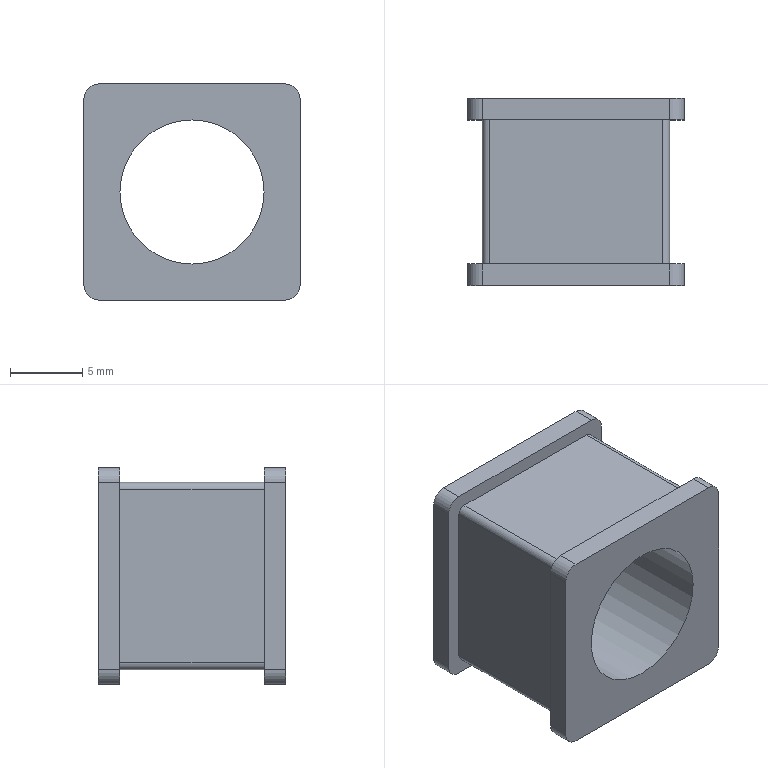Component | NX | FILLER_BLOCK | 1 solid | 29 faces | volume 1339 mm3 | plane 16 | cylinder 13 | commonest cylinder face diameters 2 x8 1 x4 10 x1